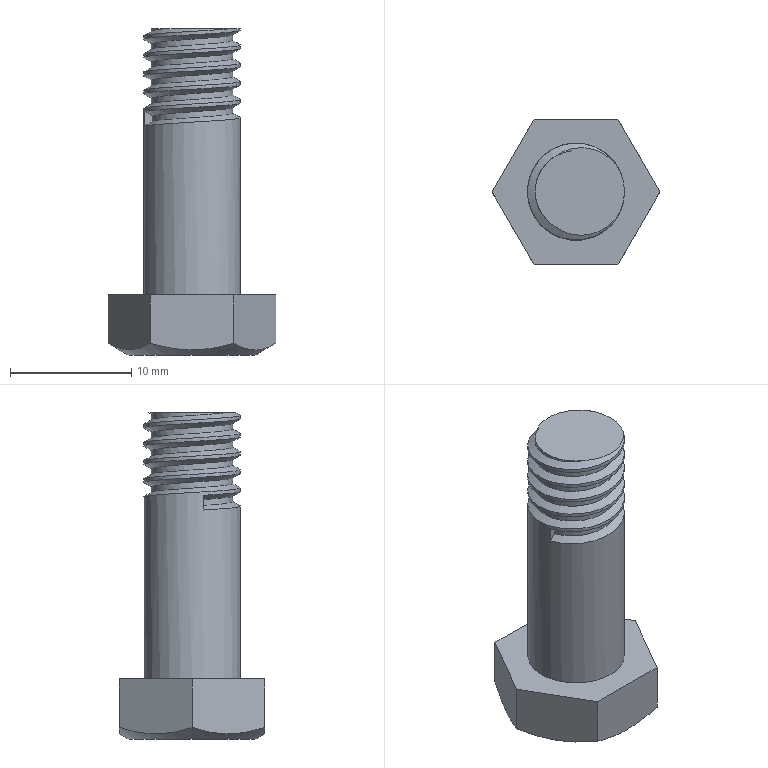Component | NX | NUT_M8X6_3 | 1 solid | 20 faces | volume 1653 mm3 | plane 10 | cylinder 7 | spline 2 | cone 1 | commonest cylinder face diameters 8 x6 6.75 x1